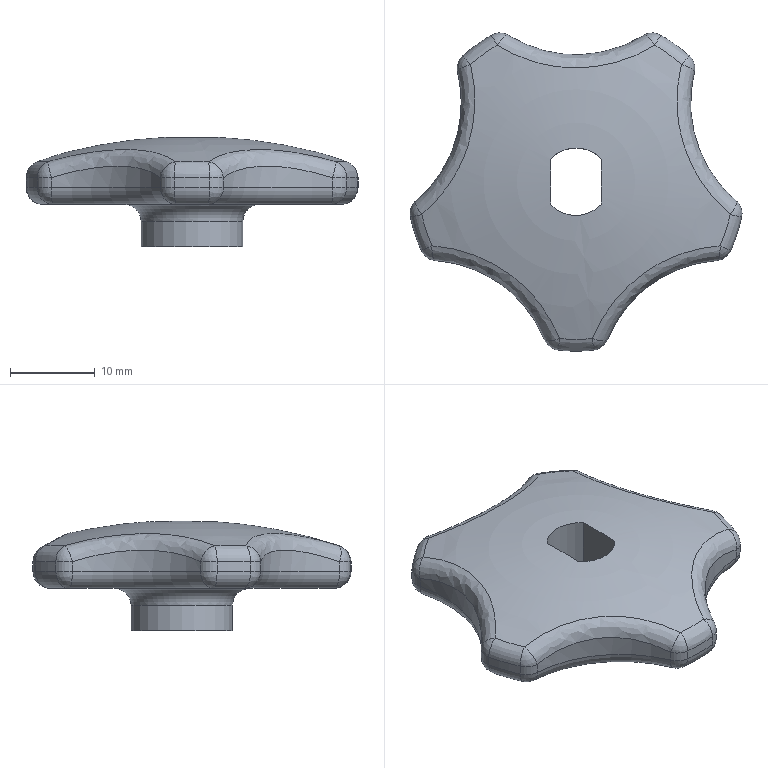Component | NX | KNOB | 1 solid | 69 faces | volume 6213 mm3 | cylinder 23 | sphere 21 | torus 16 | spline 5 | plane 4 | commonest cylinder face diameters 4 x10 40 x5 30 x5 8 x2 12 x1